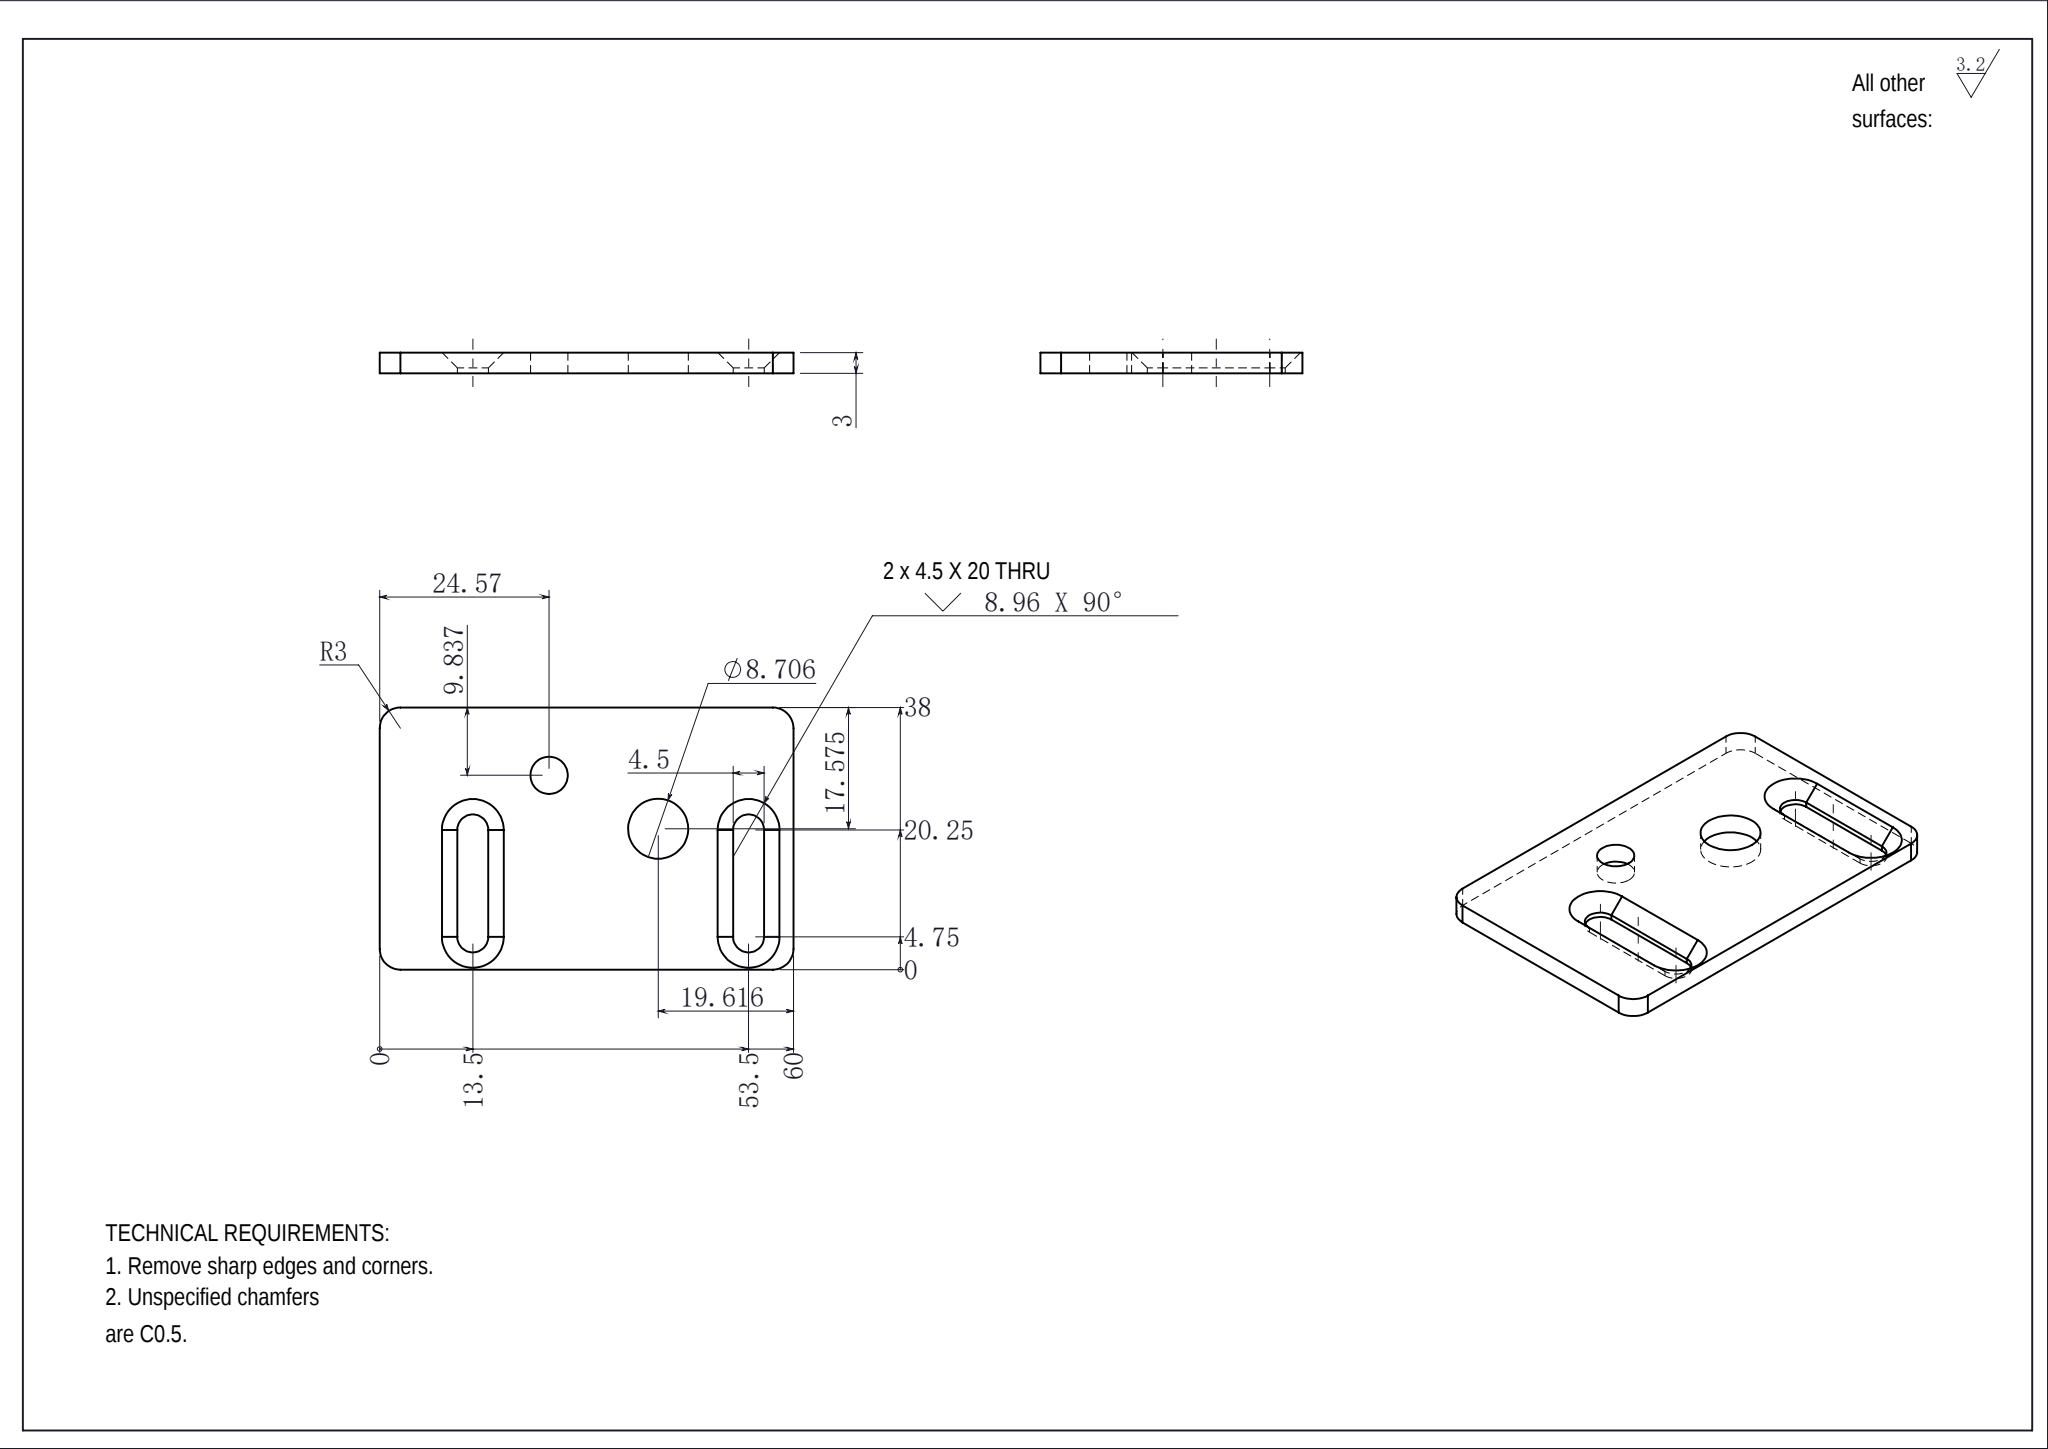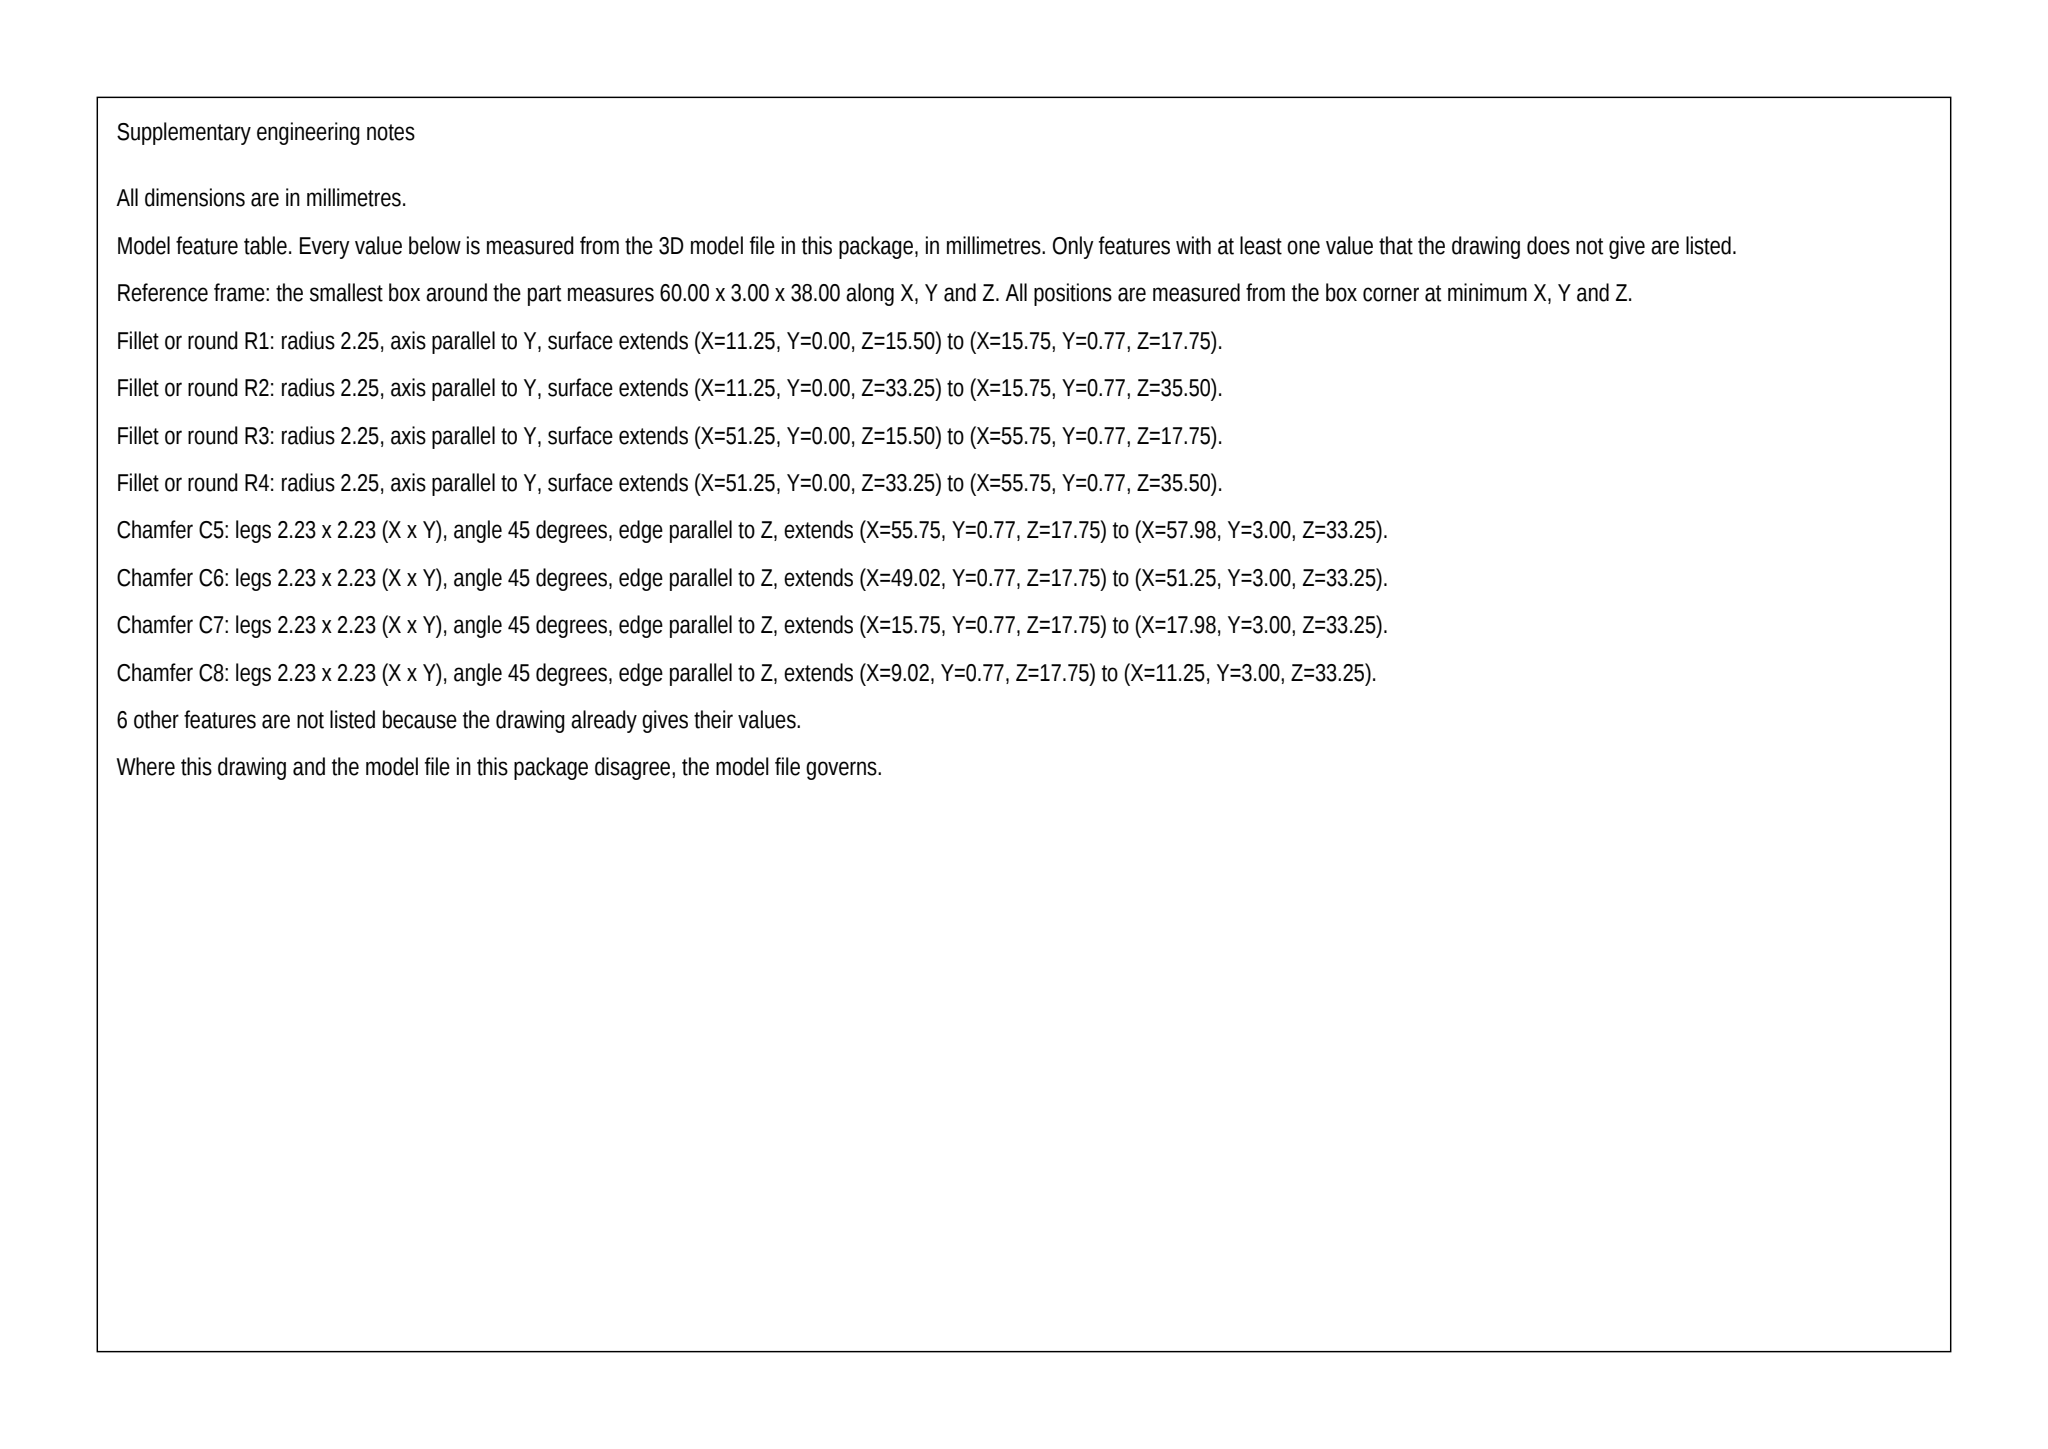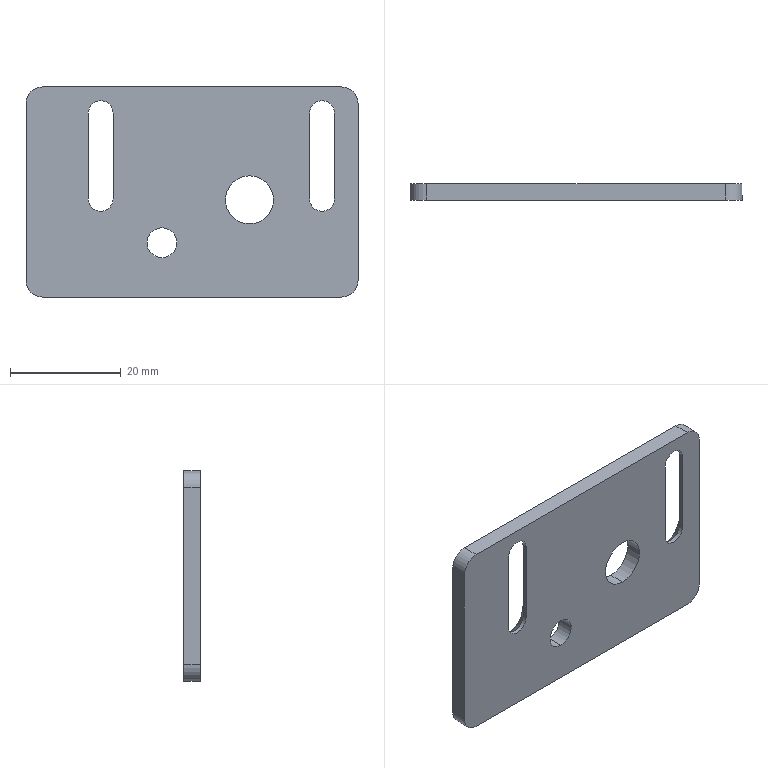Part | SolidWorks | mm | 1 solid | 34 faces | box 60 x 3 x 38 mm | volume 5808 mm3 | cylinder 14 | plane 14 | cone 6 | commonest cylinder face diameters 4.5 x6 6 x4 8.706 x2 5.409 x2